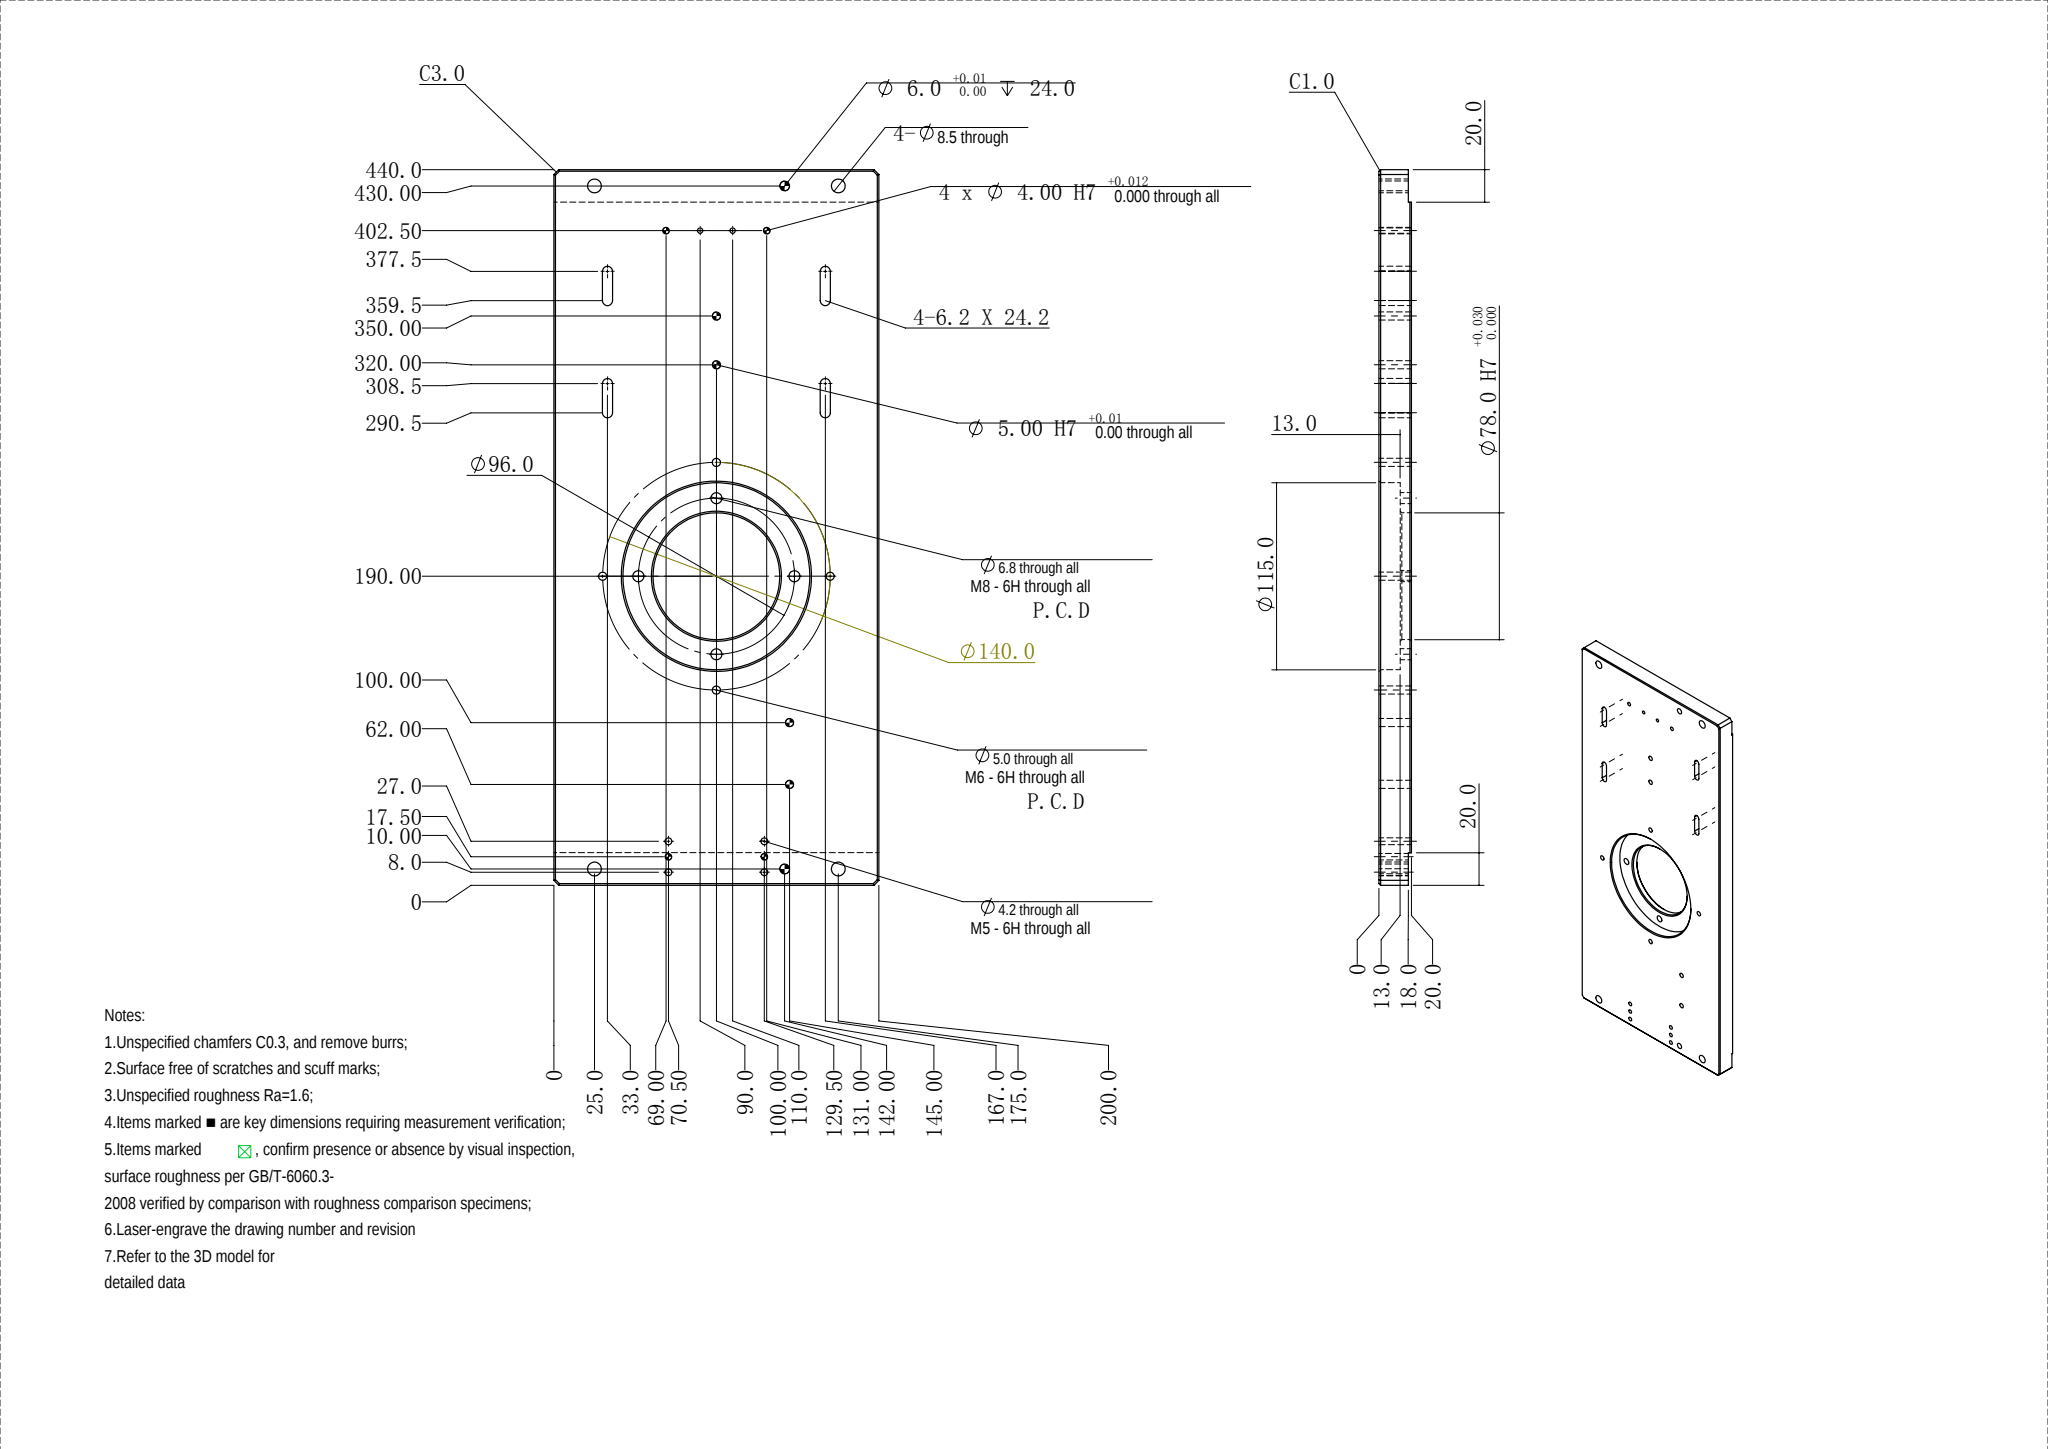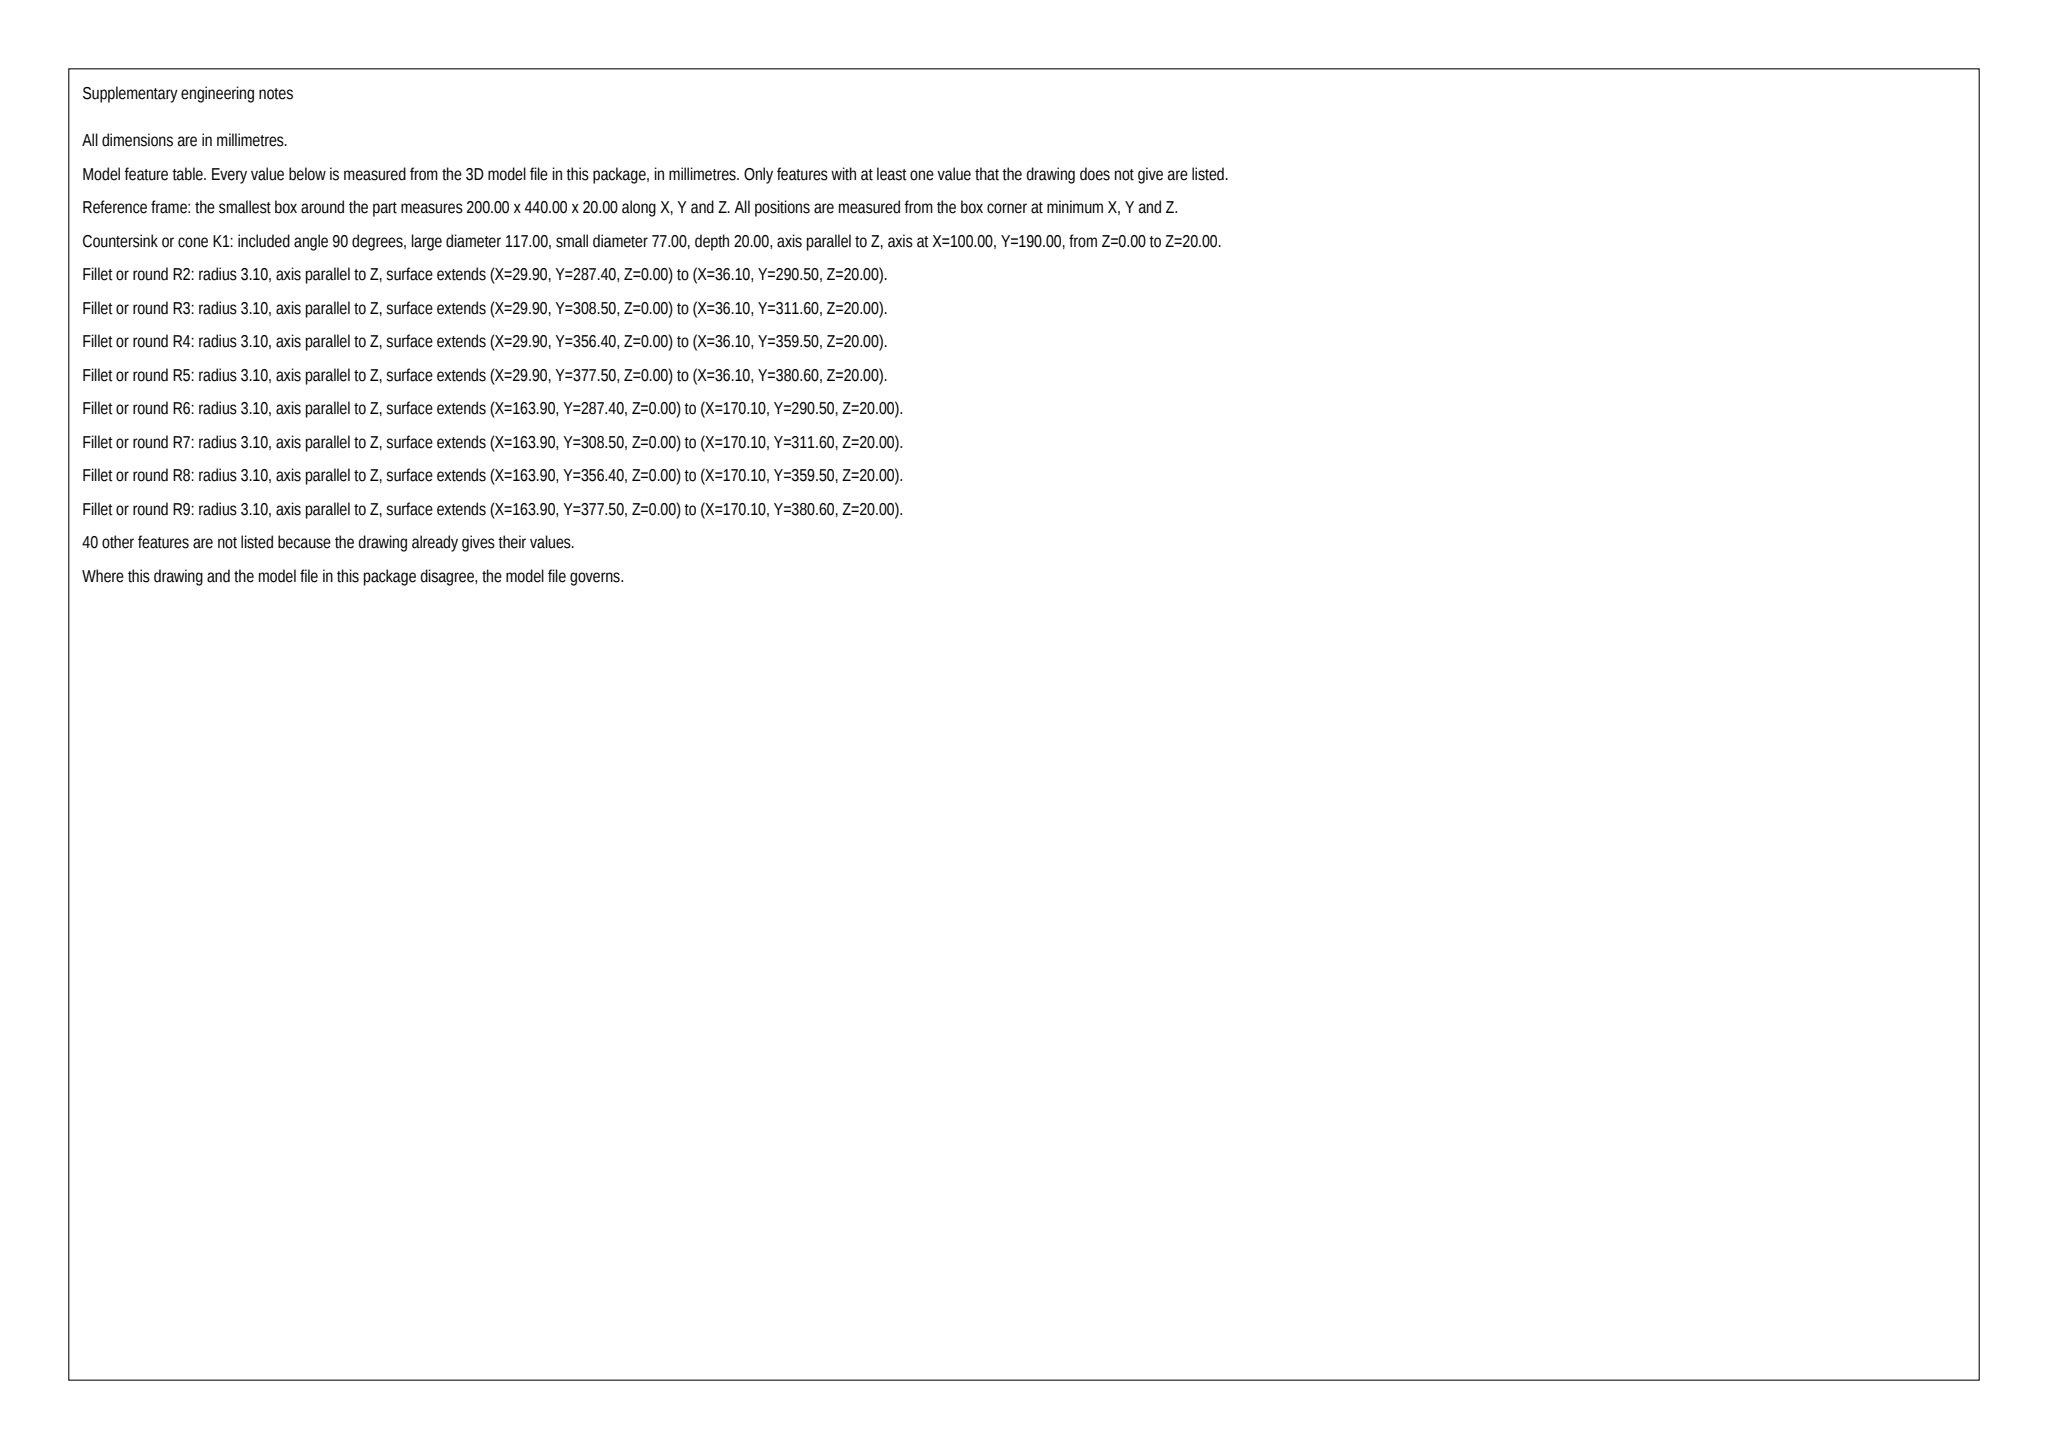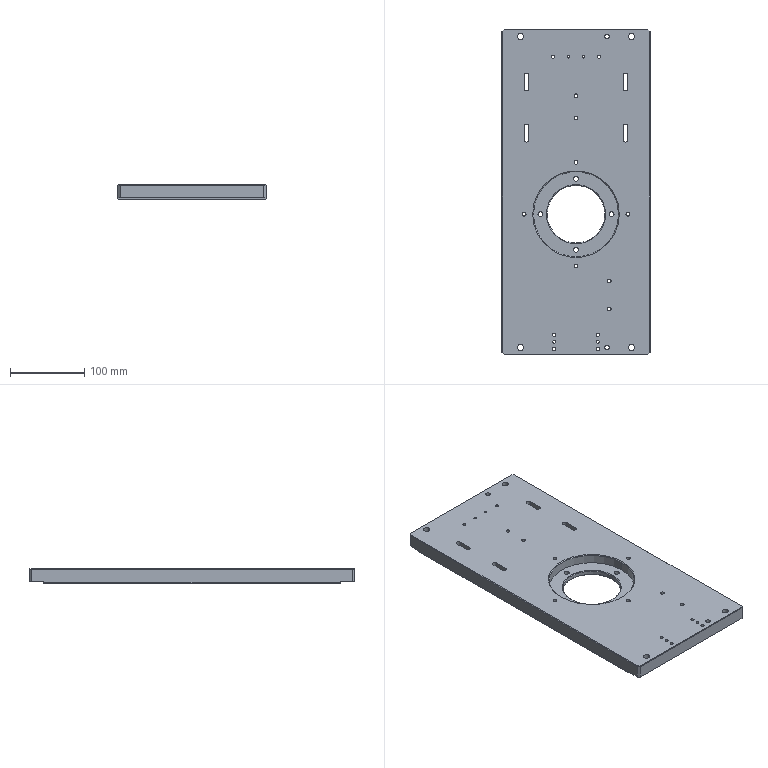Part | SolidWorks | mm | 1 solid | 107 faces | box 200 x 440 x 20 mm | volume 1550778 mm3 | cylinder 68 | plane 33 | cone 6 | commonest cylinder face diameters 5 x16 8.5 x8 4 x8 4.2 x8 6.8 x8 6.2 x8 6 x4 3.3 x4